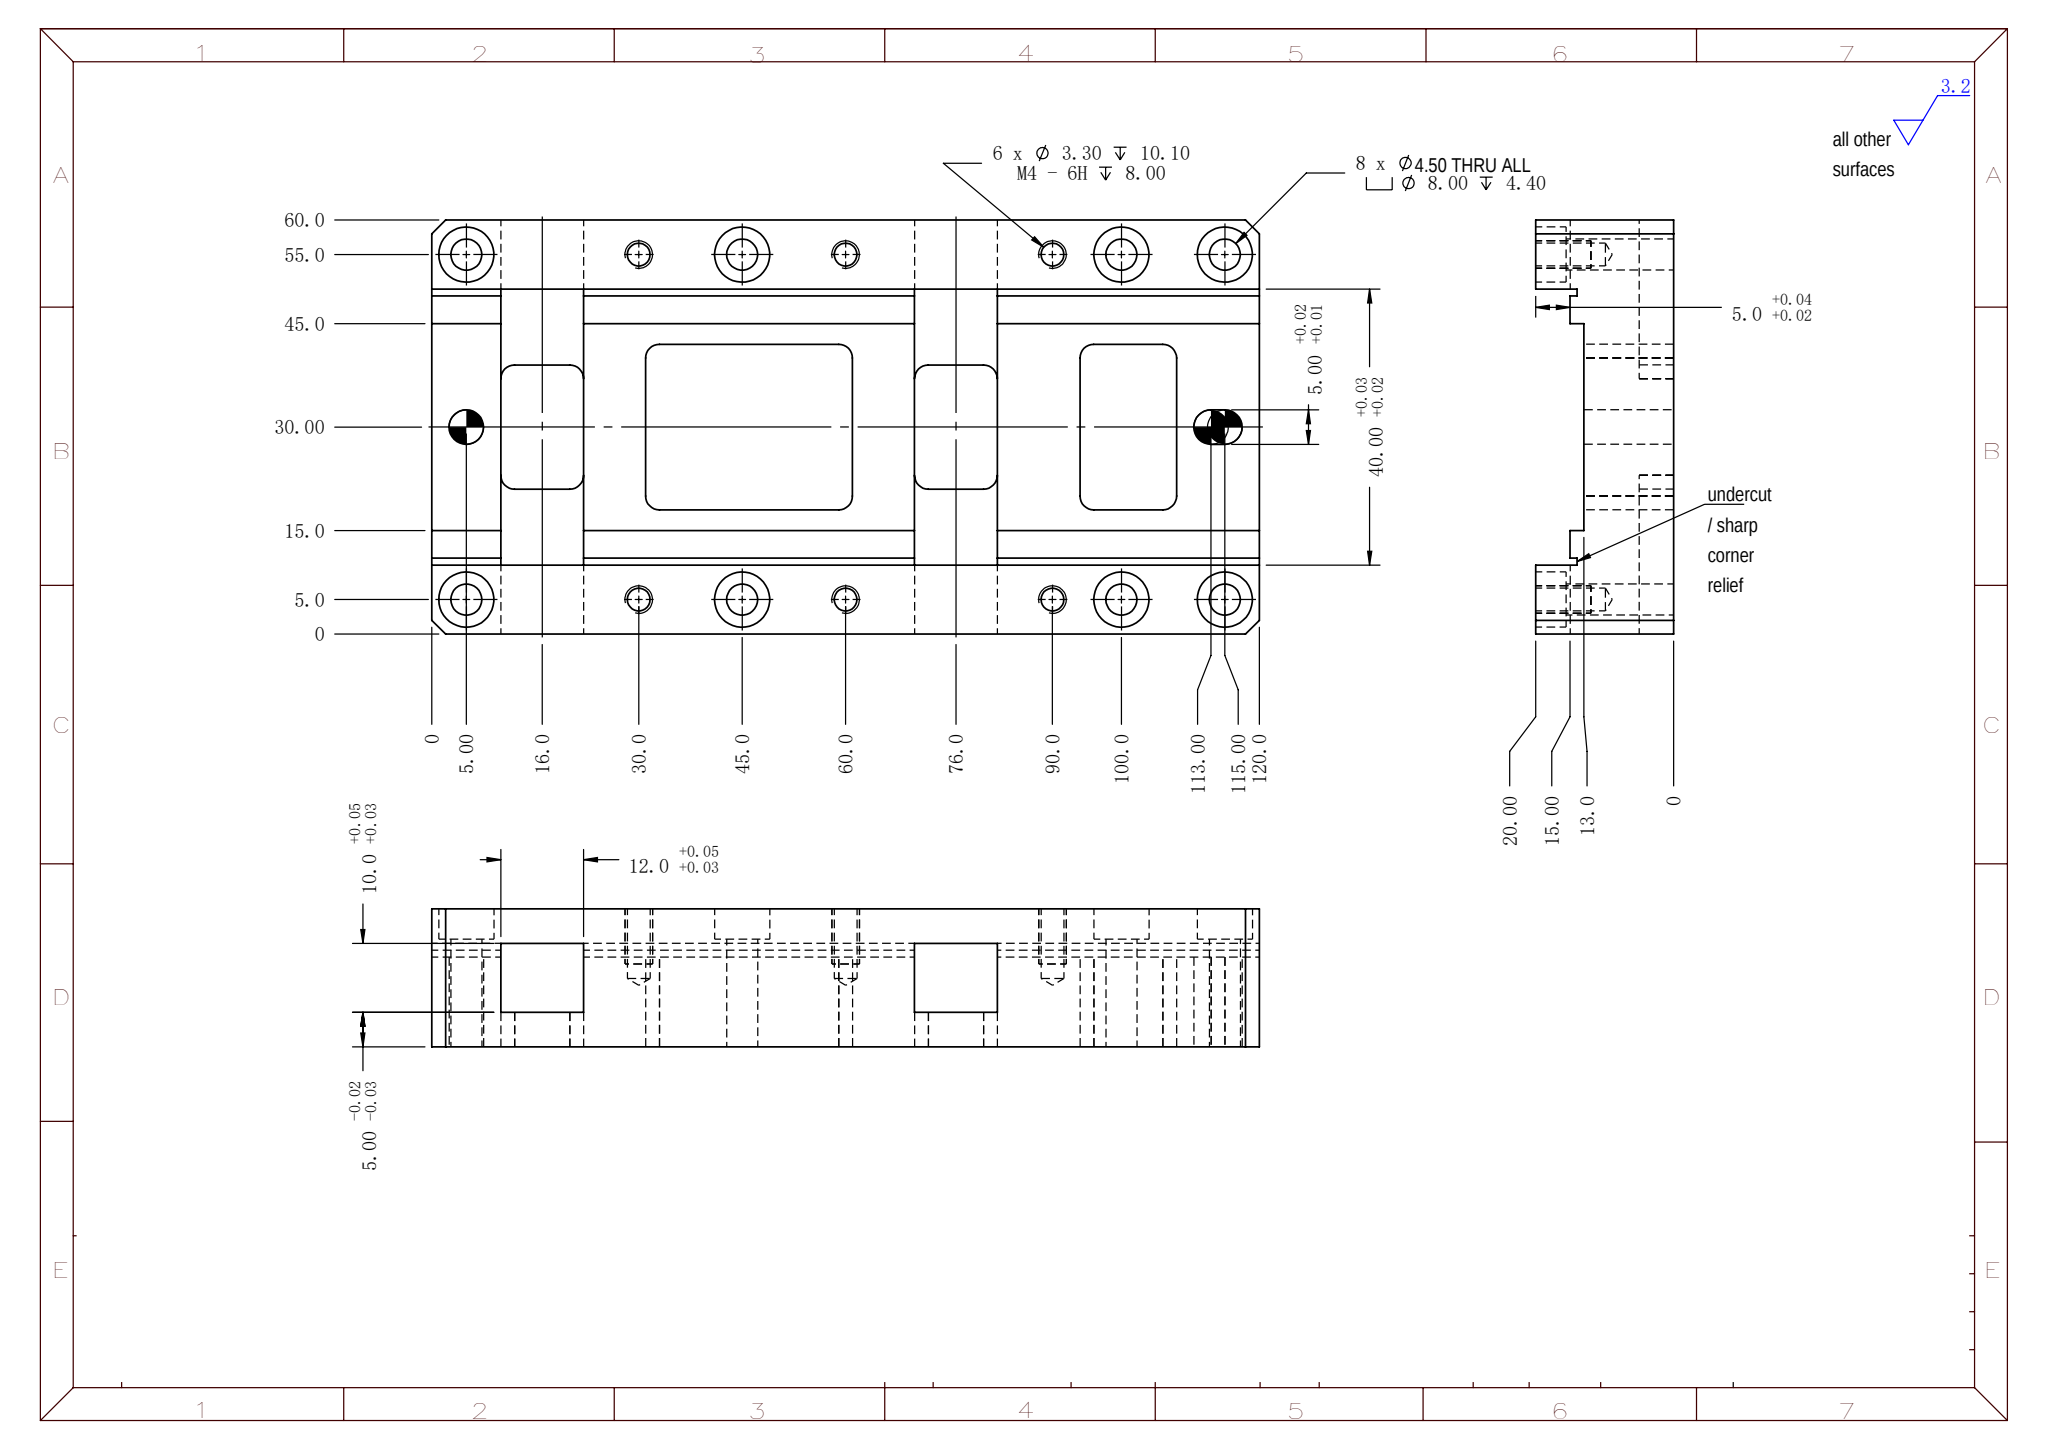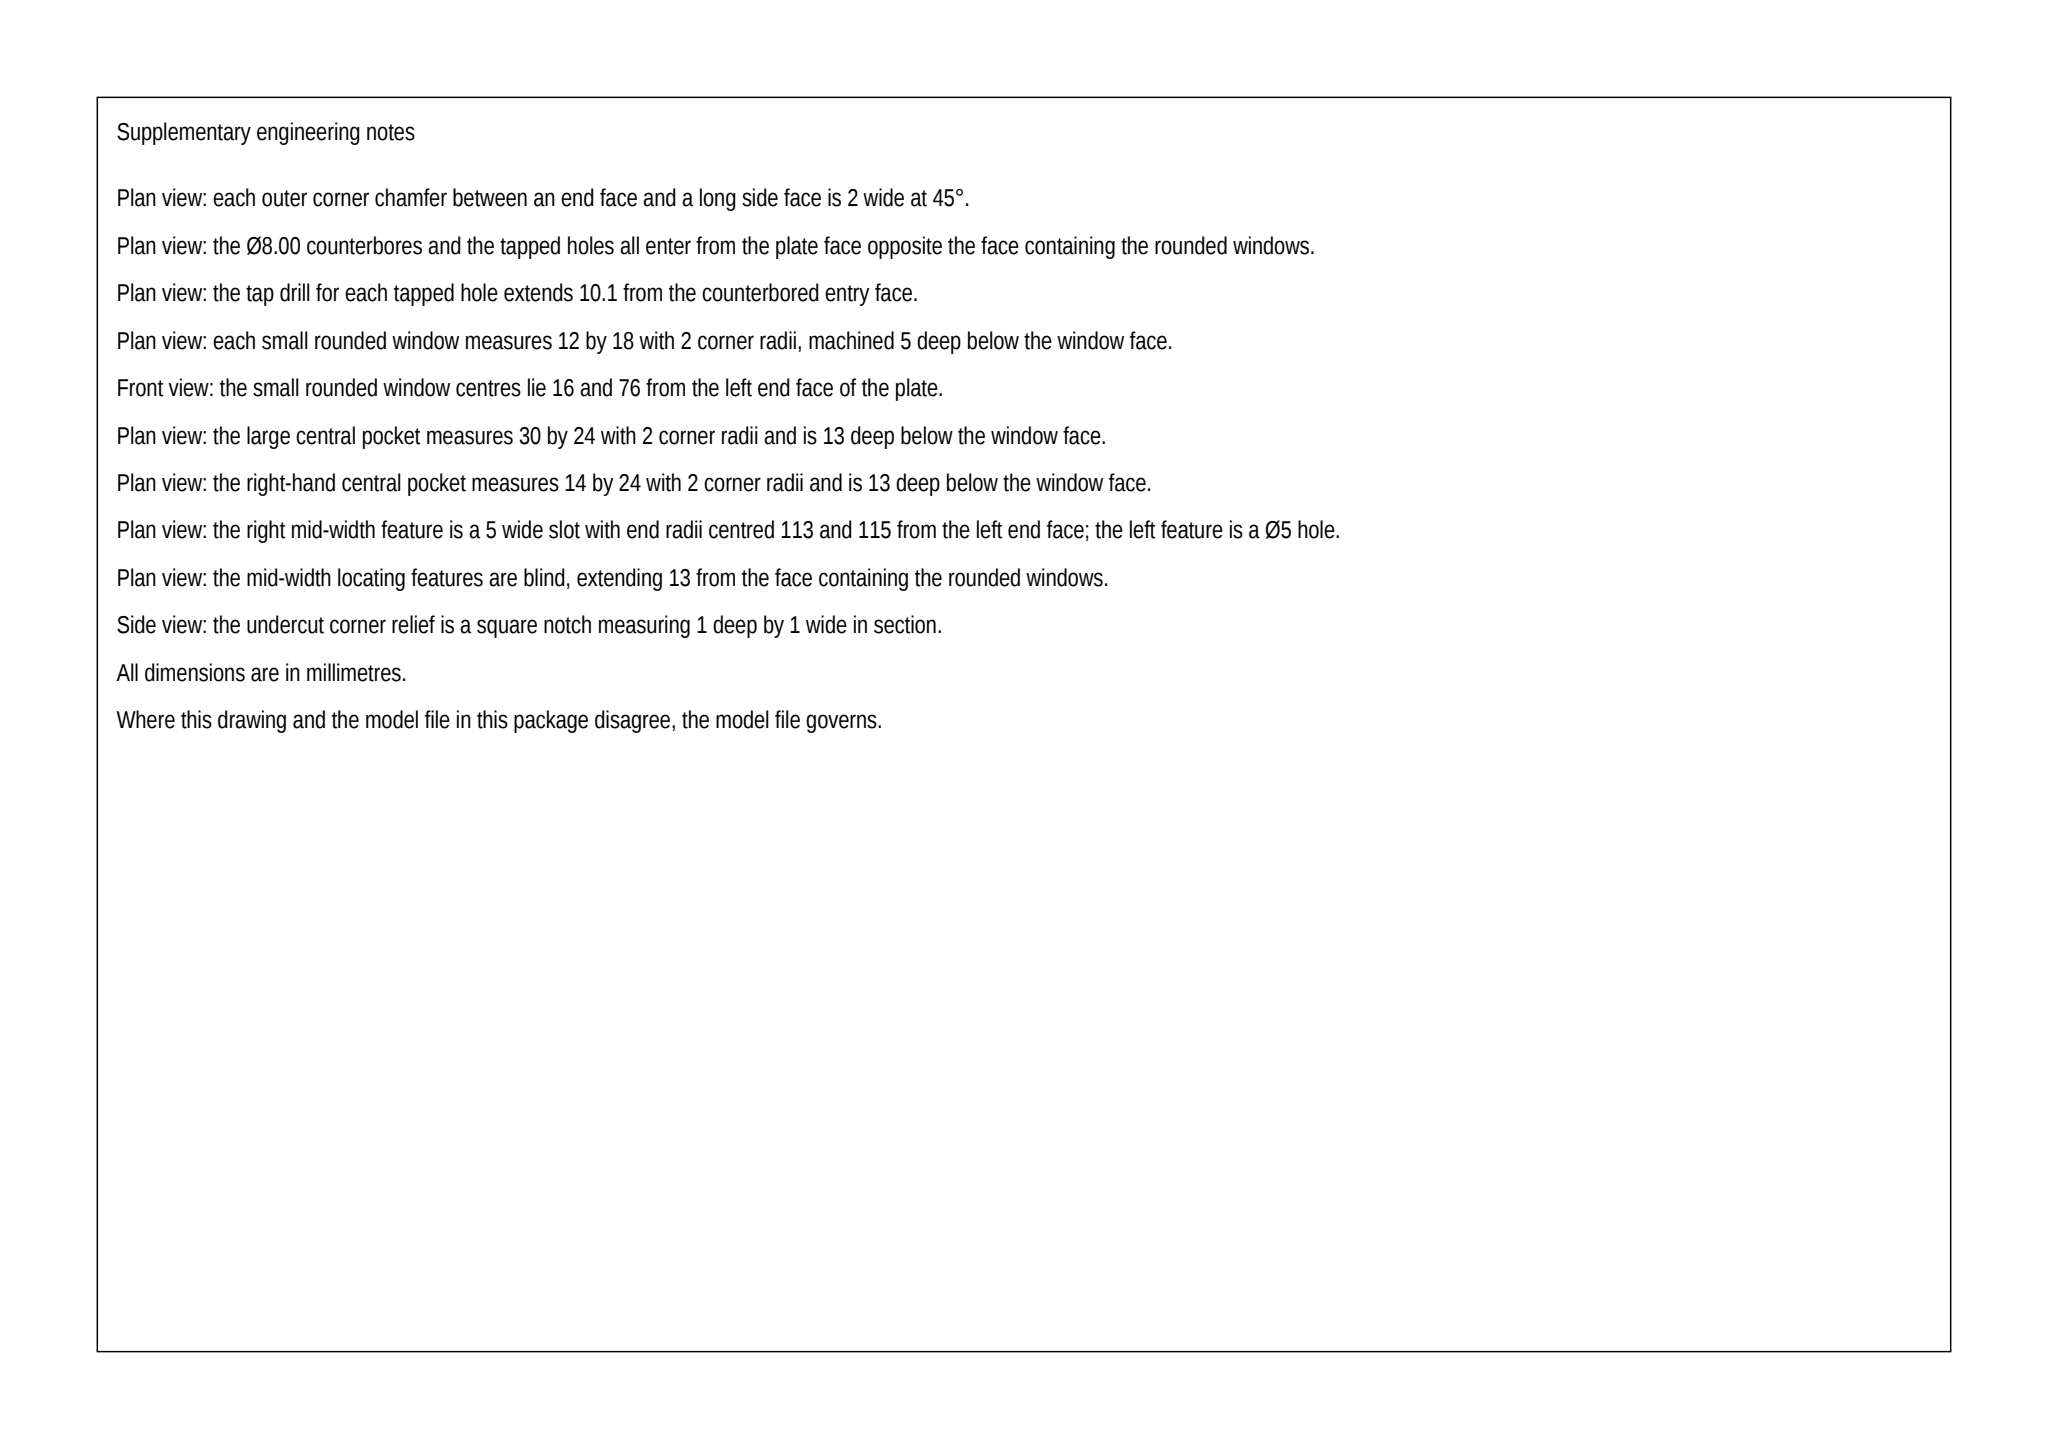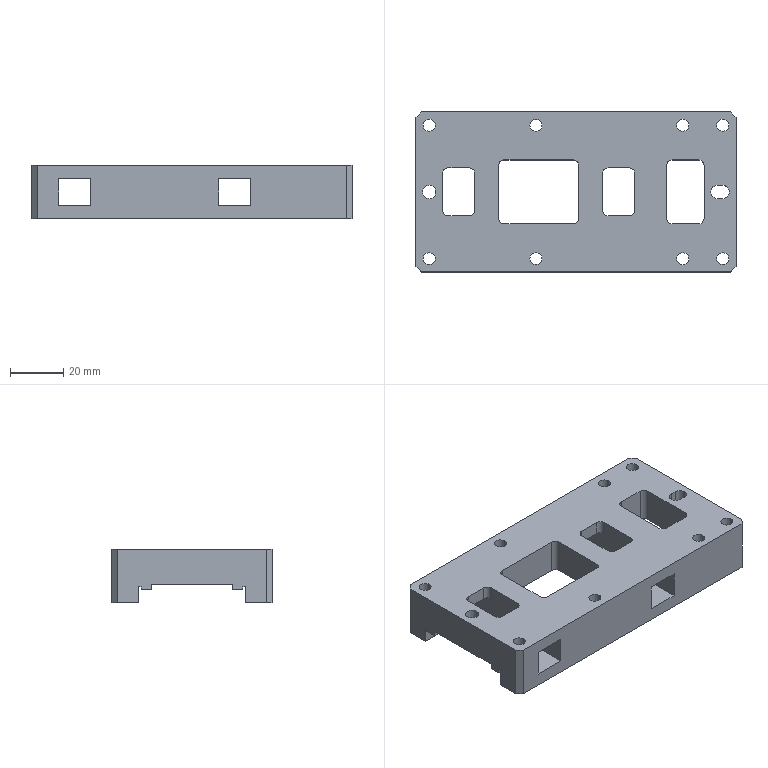Part | SolidWorks | mm | 1 solid | 151 faces | box 120 x 60 x 20 mm | volume 78794 mm3 | plane 74 | cylinder 65 | cone 12 | commonest cylinder face diameters 8 x16 4.5 x16 4 x16 3.3 x12 5 x5
Drawing notes:
ALL DIMENSIONS IN MILLIMETRES (mm). | from the solid: STEP model units mm; bbox_xyz 120.0 x 60.0 x 20.0
8X Ø4.5 THRU, C'BORE Ø8.0 DP 4.4 FROM TOP FACE (Z20); AT X=5, 45, 100, 115 AND Y=5, 55 FROM BOTTOM-LEFT CORNER (X0,Y0). | from the solid: cylinders dia 4.5 axis z len 15.6 and dia 8.0 axis z len 4.4 at (5,5),(5,55),(45,5),(45,55),(100,5),(100,55),(115,5),(115,55)
8X Ø4.0 DP 5.0; AT X=12, 20, 72, 80 AND Y=23, 37 FROM X0/Y0 CORNER. | from the solid: cylinders dia 4.0 axis z length 5.0 at (12,23),(12,37),(20,23),(20,37),(72,23),(72,37),(80,23),(80,37)
8X Ø4.0 DP 13.0; AT X=33, 59, 96, 106 AND Y=20, 40 FROM X0/Y0 CORNER. | from the solid: cylinders dia 4.0 axis z length 13.0 at (33,20),(33,40),(59,20),(59,40),(96,20),(96,40),(106,20),(106,40)
3X Ø5.00 DP 13.0 AT (X5, Y30), (X113, Y30) AND (X115, Y30) FROM X0/Y0 CORNER. | from the solid: cylinders dia 5.0 axis z length 13.0 at (5,30),(113,30),(115,30)
CENTRAL POCKET 30.0 LONG X 24.0 WIDE: WALLS AT X=31 AND X=61, Y=18 AND Y=42 FROM X0/Y0 CORNER. | from the solid: axis_planes x=31.0, x=61.0, y=18.0, y=42.0
RIGHT-HAND POCKET 14.0 LONG X 24.0 WIDE: WALLS AT X=94 AND X=108, Y=18 AND Y=42 FROM X0/Y0 CORNER. | from the solid: axis_planes x=94.0, x=108.0, y=18.0, y=42.0
ADD TO X DIMENSION STACK FROM X0 (LEFT FACE): 10, 12, 20, 22, 31, 33, 59, 61, 70, 72, 80, 82, 94, 96, 106, 108. | from the solid: axis_planes normal x at 10.0, 22.0, 31.0, 61.0, 70.0, 82.0, 94.0, 108.0 plus Ø4.0 hole axes at x=12,20,33,59,72,80,96,106
ADD TO Y DIMENSION STACK FROM Y0 (FRONT FACE): 10, 11, 18, 20, 21, 23, 37, 39, 40, 42, 49, 50. | from the solid: axis_planes normal y at 10.0, 11.0, 18.0, 21.0, 39.0, 42.0, 49.0, 50.0 plus Ø4.0 hole axes at y=20,23,37,40
ADD TO END-VIEW HEIGHT STACK FROM BOTTOM FACE Z0: 4.4, 5.0, 6.0, 7.0 (STEP/RAIL FACE LEVELS); TOP FACE Z=20.0. | from the solid: axis_planes normal z at 0.0, 4.4, 5.0, 6.0, 7.0, 15.0, 20.0
TRANSVERSE SLOT WALLS: LEFT SLOT BETWEEN X=10 AND X=22; RIGHT SLOT BETWEEN X=70 AND X=82, FROM X0. | from the solid: axis_planes normal x at 10.0, 22.0, 70.0, 82.0
6X Ø3.30 DRILL DP 10.10 TAP M4-6H DP 8.00 AT X=30, 60, 90 AND Y=5, 55 FROM X0/Y0 CORNER (DRILL POINT 118°). | from the solid: cylinders dia 3.3 axis z len 10.1 at (30,5),(30,55),(60,5),(60,55),(90,5),(90,55); cones 118.0 ref_dia 3.3
Pocket and rib walls lie on Y = 11.0, 15.0, 18.0, 21.0, 27.5, 32.5, 39.0, 42.0, 45.0, 49.0 and 50.0 from the Y datum (Y=0 edge) | from the solid: axis_planes normal y at 11.0, 15.0, 18.0, 21.0, 27.5, 32.5, 39.0, 42.0, 45.0, 49.0, 50.0
Transverse cut-outs bounded by X=10.0 to 22.0 and X=70.0 to 82.0; floor at Z=5.0 (15.0 below top face Z=20.0) | from the solid: axis_planes x at 10.0, 22.0, 70.0, 82.0 and z at 5.0 (10 faces); bbox height 20.0
Internal step/rail faces at Z=6.0, Z=7.0 and Z=15.0 measured from bottom face Z=0 | from the solid: axis_planes normal z at 6.0 (6 faces), 7.0 (3 faces), 15.0 (4 faces)
CENTRAL RELIEF GROOVE 5.0 WIDE: WALLS AT Y=27.5 AND Y=32.5 FROM Y0 DATUM (CENTRED ON Y=30.0) | from the solid: axis_planes normal y, offsets 27.5 and 32.5 (1 face each)
build123d program:
from build123d import *

# Parameters (mm, degrees)
SKETCH1_W                                       = 120
SKETCH1_H                                       = 60
BOSS_EXTRUDE1_DEPTH                             = 10
SKETCH2_W                                       = 12
SKETCH2_H                                       = 10
CUT_EXTRUDE1_DEPTH                              = 86.44
SKETCH3_W                                       = 120
SKETCH3_H                                       = 40
CUT_EXTRUDE2_DEPTH                              = 5
CUT_EXTRUDE3_DEPTH                              = 71
M4_TAPPED_HOLE1_D                               = 3.3
M4_TAPPED_HOLE1_DEPTH                           = 10.1
M4_TAPPED_HOLE1_TIP                             = 0.9914
SKETCH8_W                                       = 120
SKETCH8_H                                       = 1
CUT_EXTRUDE4_DEPTH                              = 1
M4_HEX_SOCKET_HEAD_CAP_SCREW_CBORE1_D           = 4.5
M4_HEX_SOCKET_HEAD_CAP_SCREW_CBORE1_CBORE_D     = 8
M4_HEX_SOCKET_HEAD_CAP_SCREW_CBORE1_CBORE_DEPTH = 4.4
CUT_EXTRUDE6_DEPTH                              = 69.739
SIZE_MM_DOWEL_PIN_HOLE1_D                       = 5
CUT_EXTRUDE7_DEPTH                              = 71
CHAMFER1_SIZE                                   = 2
SKETCH17_W                                      = 120
SKETCH17_H                                      = 30
CUT_EXTRUDE8_DEPTH                              = 2


with BuildPart() as part:
    # Sketch1 → Boss-Extrude1 (new, symmetric)
    with BuildSketch(Plane.XY):
        Rectangle(SKETCH1_W, SKETCH1_H)
    extrude(amount=BOSS_EXTRUDE1_DEPTH, both=True)

    # Sketch2 → Cut-Extrude1 (cut, through all)
    with BuildSketch(Plane(origin=(0, 30, 0), x_dir=(1, 0, 0), z_dir=(0, 1, 0))):
        with Locations((-44, 0)):
            Rectangle(SKETCH2_W, SKETCH2_H)
        with Locations((16, 0)):
            Rectangle(SKETCH2_W, SKETCH2_H)
    extrude(amount=-CUT_EXTRUDE1_DEPTH, mode=Mode.SUBTRACT)

    # Sketch3 → Cut-Extrude2 (cut)
    with BuildSketch(Plane(origin=(0, 0, -10), x_dir=(-1, 0, 0), z_dir=(0, 0, -1))):
        Rectangle(SKETCH3_W, SKETCH3_H)
    extrude(amount=-CUT_EXTRUDE2_DEPTH, mode=Mode.SUBTRACT)

    # Sketch4 → Cut-Extrude3 (cut, through all)
    with BuildSketch(Plane.XY.offset(10)):
        with BuildLine():
            Line((-48, -9), (-40, -9))
            ThreePointArc((-40, -9), (-38.586, -8.414), (-38, -7))
            Line((-38, -7), (-38, 7))
            ThreePointArc((-38, 7), (-38.586, 8.414), (-40, 9))
            Line((-40, 9), (-48, 9))
            ThreePointArc((-48, 9), (-49.414, 8.414), (-50, 7))
            Line((-50, 7), (-50, -7))
            ThreePointArc((-50, -7), (-49.414, -8.414), (-48, -9))
        make_face()
        with BuildLine():
            Line((12, -9), (20, -9))
            ThreePointArc((20, -9), (21.414, -8.414), (22, -7))
            Line((22, -7), (22, 7))
            ThreePointArc((22, 7), (21.414, 8.414), (20, 9))
            Line((20, 9), (12, 9))
            ThreePointArc((12, 9), (10.586, 8.414), (10, 7))
            Line((10, 7), (10, -7))
            ThreePointArc((10, -7), (10.586, -8.414), (12, -9))
        make_face()
    extrude(amount=-CUT_EXTRUDE3_DEPTH, mode=Mode.SUBTRACT)

    # M4 Tapped Hole1
    with Locations(Plane(origin=(0, 0, -10), x_dir=(-1, 0, 0), z_dir=(0, 0, -1))):
        with Locations((-30, 25), (0, 25), (30, 25), (-30, -25), (0, -25), (30, -25)):
            Hole(M4_TAPPED_HOLE1_D / 2, depth=M4_TAPPED_HOLE1_DEPTH)
            with Locations((0, 0, -(M4_TAPPED_HOLE1_DEPTH + M4_TAPPED_HOLE1_TIP / 2))):  # 118° drill point
                Cone(0, M4_TAPPED_HOLE1_D / 2, M4_TAPPED_HOLE1_TIP, mode=Mode.SUBTRACT)

    # Sketch8 → Cut-Extrude4 (cut)
    with BuildSketch(Plane(origin=(0, 0, -5), x_dir=(-1, 0, 0), z_dir=(0, 0, -1))):
        with Locations((0, 19.5)):
            Rectangle(SKETCH8_W, SKETCH8_H)
        with Locations((0, -19.5)):
            Rectangle(SKETCH8_W, SKETCH8_H)
    extrude(amount=-CUT_EXTRUDE4_DEPTH, mode=Mode.SUBTRACT)

    # M4 Hex Socket Head Cap Screw CBORE1 (through all)
    with Locations(Plane(origin=(0, 0, -10), x_dir=(-1, 0, 0), z_dir=(0, 0, -1))):
        with Locations((-55, 25), (15, 25), (55, 25), (-40, 25), (-40, -25), (55, -25), (15, -25), (-55, -25)):
            CounterBoreHole(M4_HEX_SOCKET_HEAD_CAP_SCREW_CBORE1_D / 2, M4_HEX_SOCKET_HEAD_CAP_SCREW_CBORE1_CBORE_D / 2, M4_HEX_SOCKET_HEAD_CAP_SCREW_CBORE1_CBORE_DEPTH)

    # Sketch12 → Cut-Extrude6 (cut, through all)
    with BuildSketch(Plane(origin=(0, 0, -5), x_dir=(-1, 0, 0), z_dir=(0, 0, -1))):
        with BuildLine():
            Line((-46, -12), (-36, -12))
            ThreePointArc((-36, -12), (-34.586, -11.414), (-34, -10))
            Line((-34, -10), (-34, 10))
            ThreePointArc((-34, 10), (-34.586, 11.414), (-36, 12))
            Line((-36, 12), (-46, 12))
            ThreePointArc((-46, 12), (-47.414, 11.414), (-48, 10))
            Line((-48, 10), (-48, -10))
            ThreePointArc((-48, -10), (-47.414, -11.414), (-46, -12))
        make_face()
        with BuildLine():
            Line((1, -12), (27, -12))
            ThreePointArc((27, -12), (28.414, -11.414), (29, -10))
            Line((29, -10), (29, 10))
            ThreePointArc((29, 10), (28.414, 11.414), (27, 12))
            Line((27, 12), (1, 12))
            ThreePointArc((1, 12), (-0.4142, 11.414), (-1, 10))
            Line((-1, 10), (-1, -10))
            ThreePointArc((-1, -10), (-0.4142, -11.414), (1, -12))
        make_face()
    extrude(amount=-CUT_EXTRUDE6_DEPTH, mode=Mode.SUBTRACT)

    # Size mm Dowel Pin Hole1 (through all)
    with Locations(Plane.XY.offset(10)):
        with Locations((-55, 0), (54, 0)):
            Hole(SIZE_MM_DOWEL_PIN_HOLE1_D / 2)

    # Sketch16 → Cut-Extrude7 (cut, through all)
    with BuildSketch(Plane.XY.offset(10)):
        with BuildLine():
            Line((53, 2.5), (55, 2.5))
            ThreePointArc((55, 2.5), (57.5, 0), (55, -2.5))
            Line((55, -2.5), (53, -2.5))
            ThreePointArc((53, -2.5), (50.5, 0), (53, 2.5))
        make_face()
    extrude(amount=-CUT_EXTRUDE7_DEPTH, mode=Mode.SUBTRACT)

    # Chamfer1
    chamfer1_edges = [part.edges().sort_by_distance(p)[0] for p in [
        (60, -30, 0),
        (-60, -30, 0),
        (-60, 30, 0),
        (60, 30, 0),
    ]]
    chamfer(chamfer1_edges, length=CHAMFER1_SIZE)

    # Sketch17 → Cut-Extrude8 (cut)
    with BuildSketch(Plane(origin=(0, 0, -5), x_dir=(-1, 0, 0), z_dir=(0, 0, -1))):
        Rectangle(SKETCH17_W, SKETCH17_H)
    extrude(amount=-CUT_EXTRUDE8_DEPTH, mode=Mode.SUBTRACT)


solid = part.part